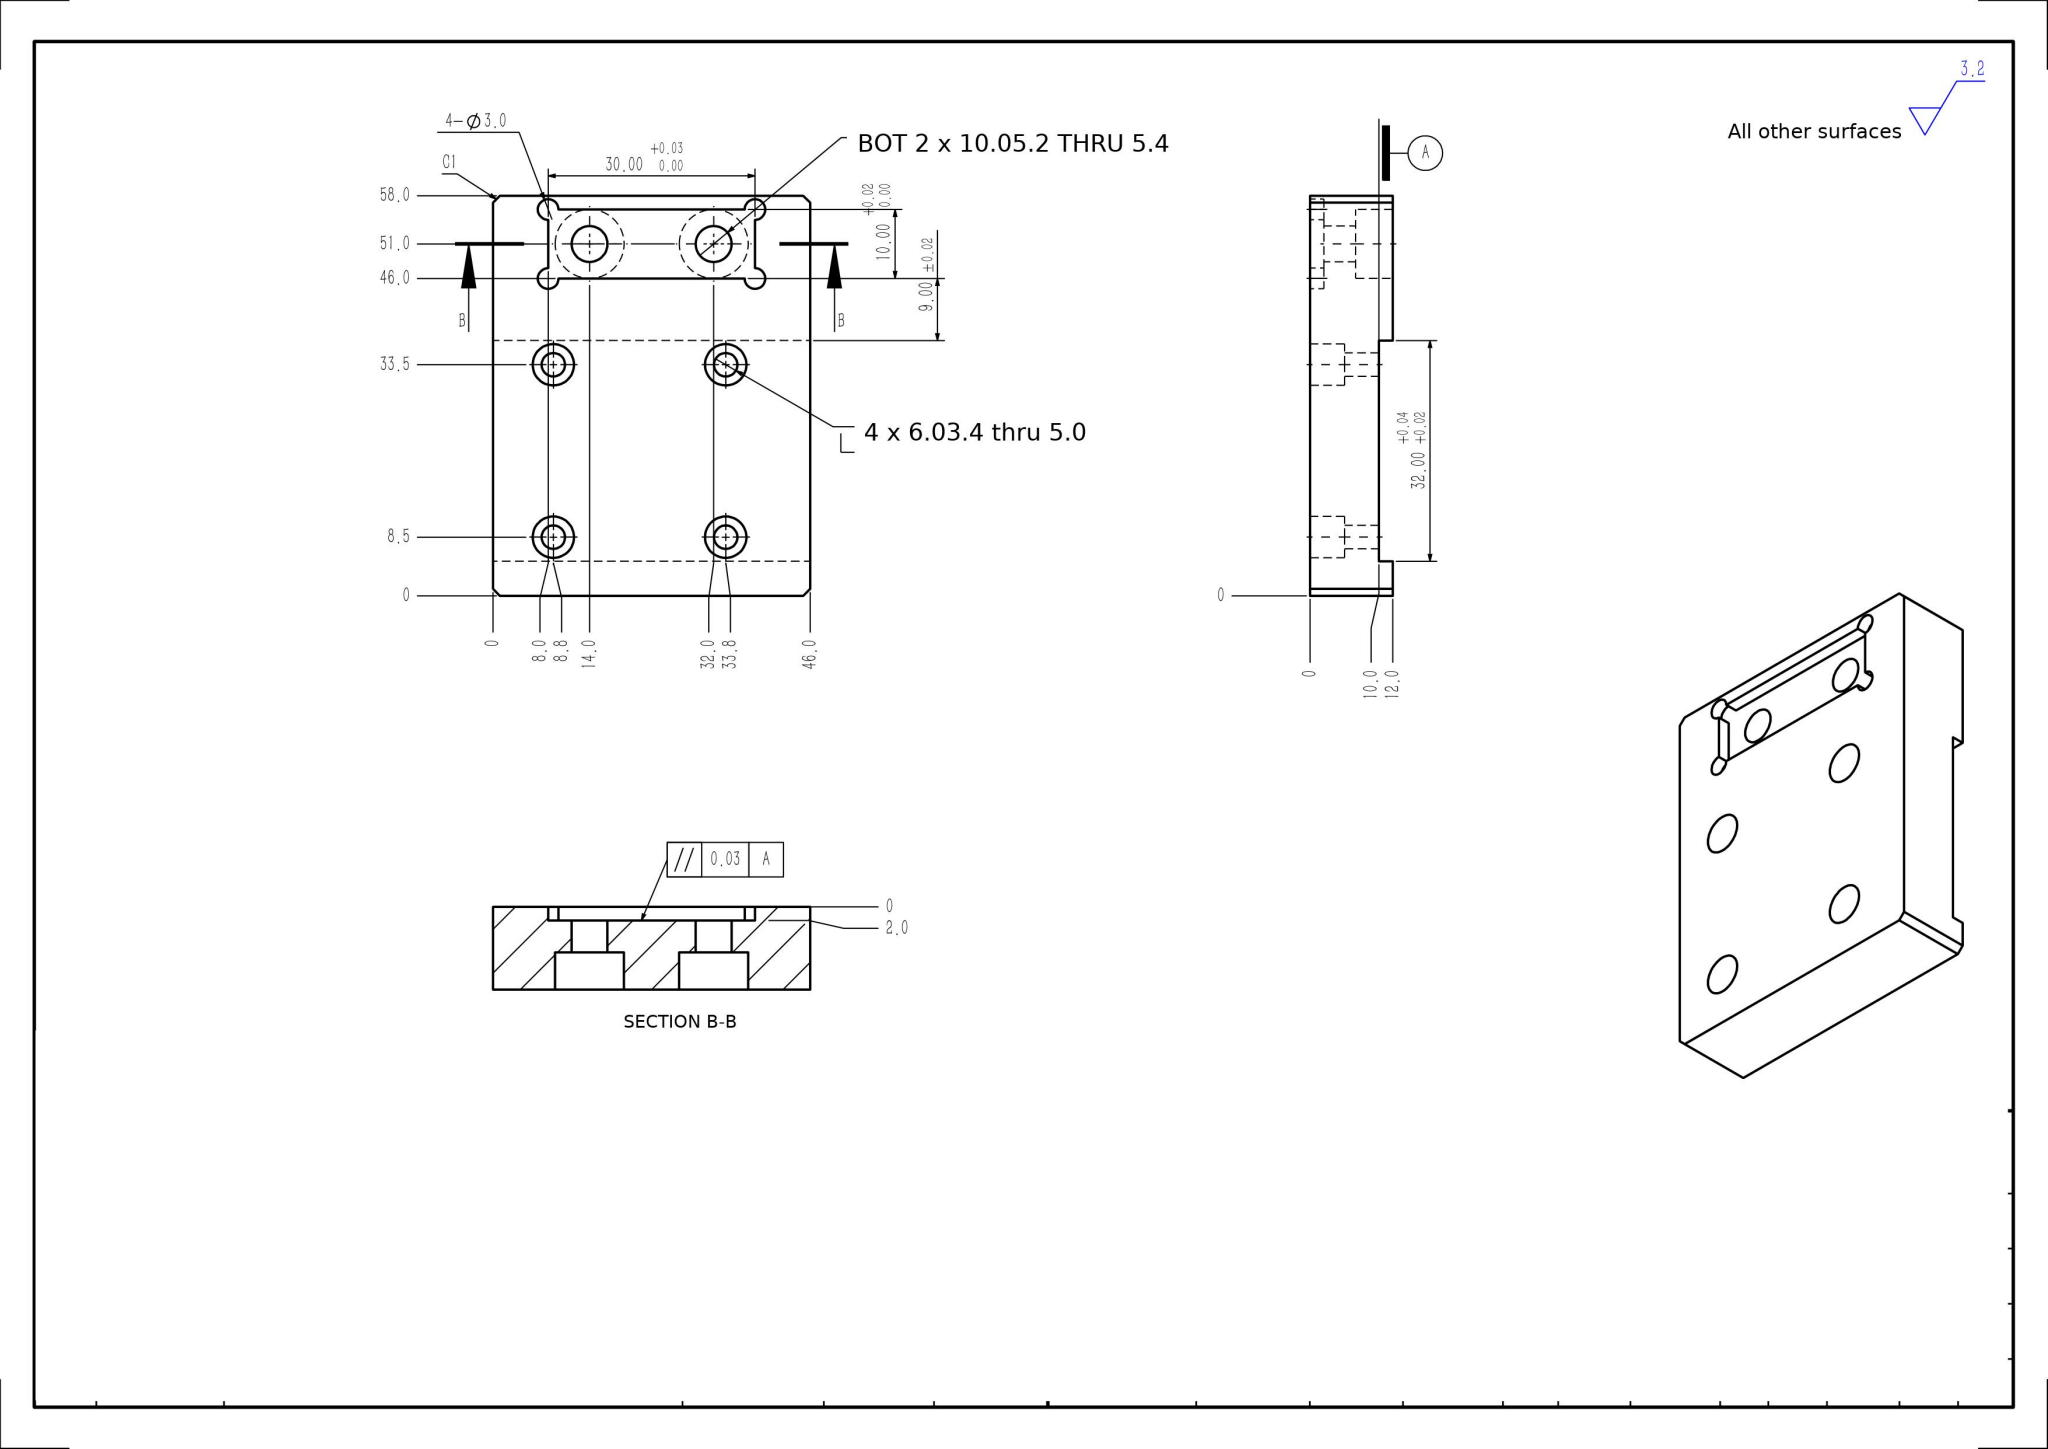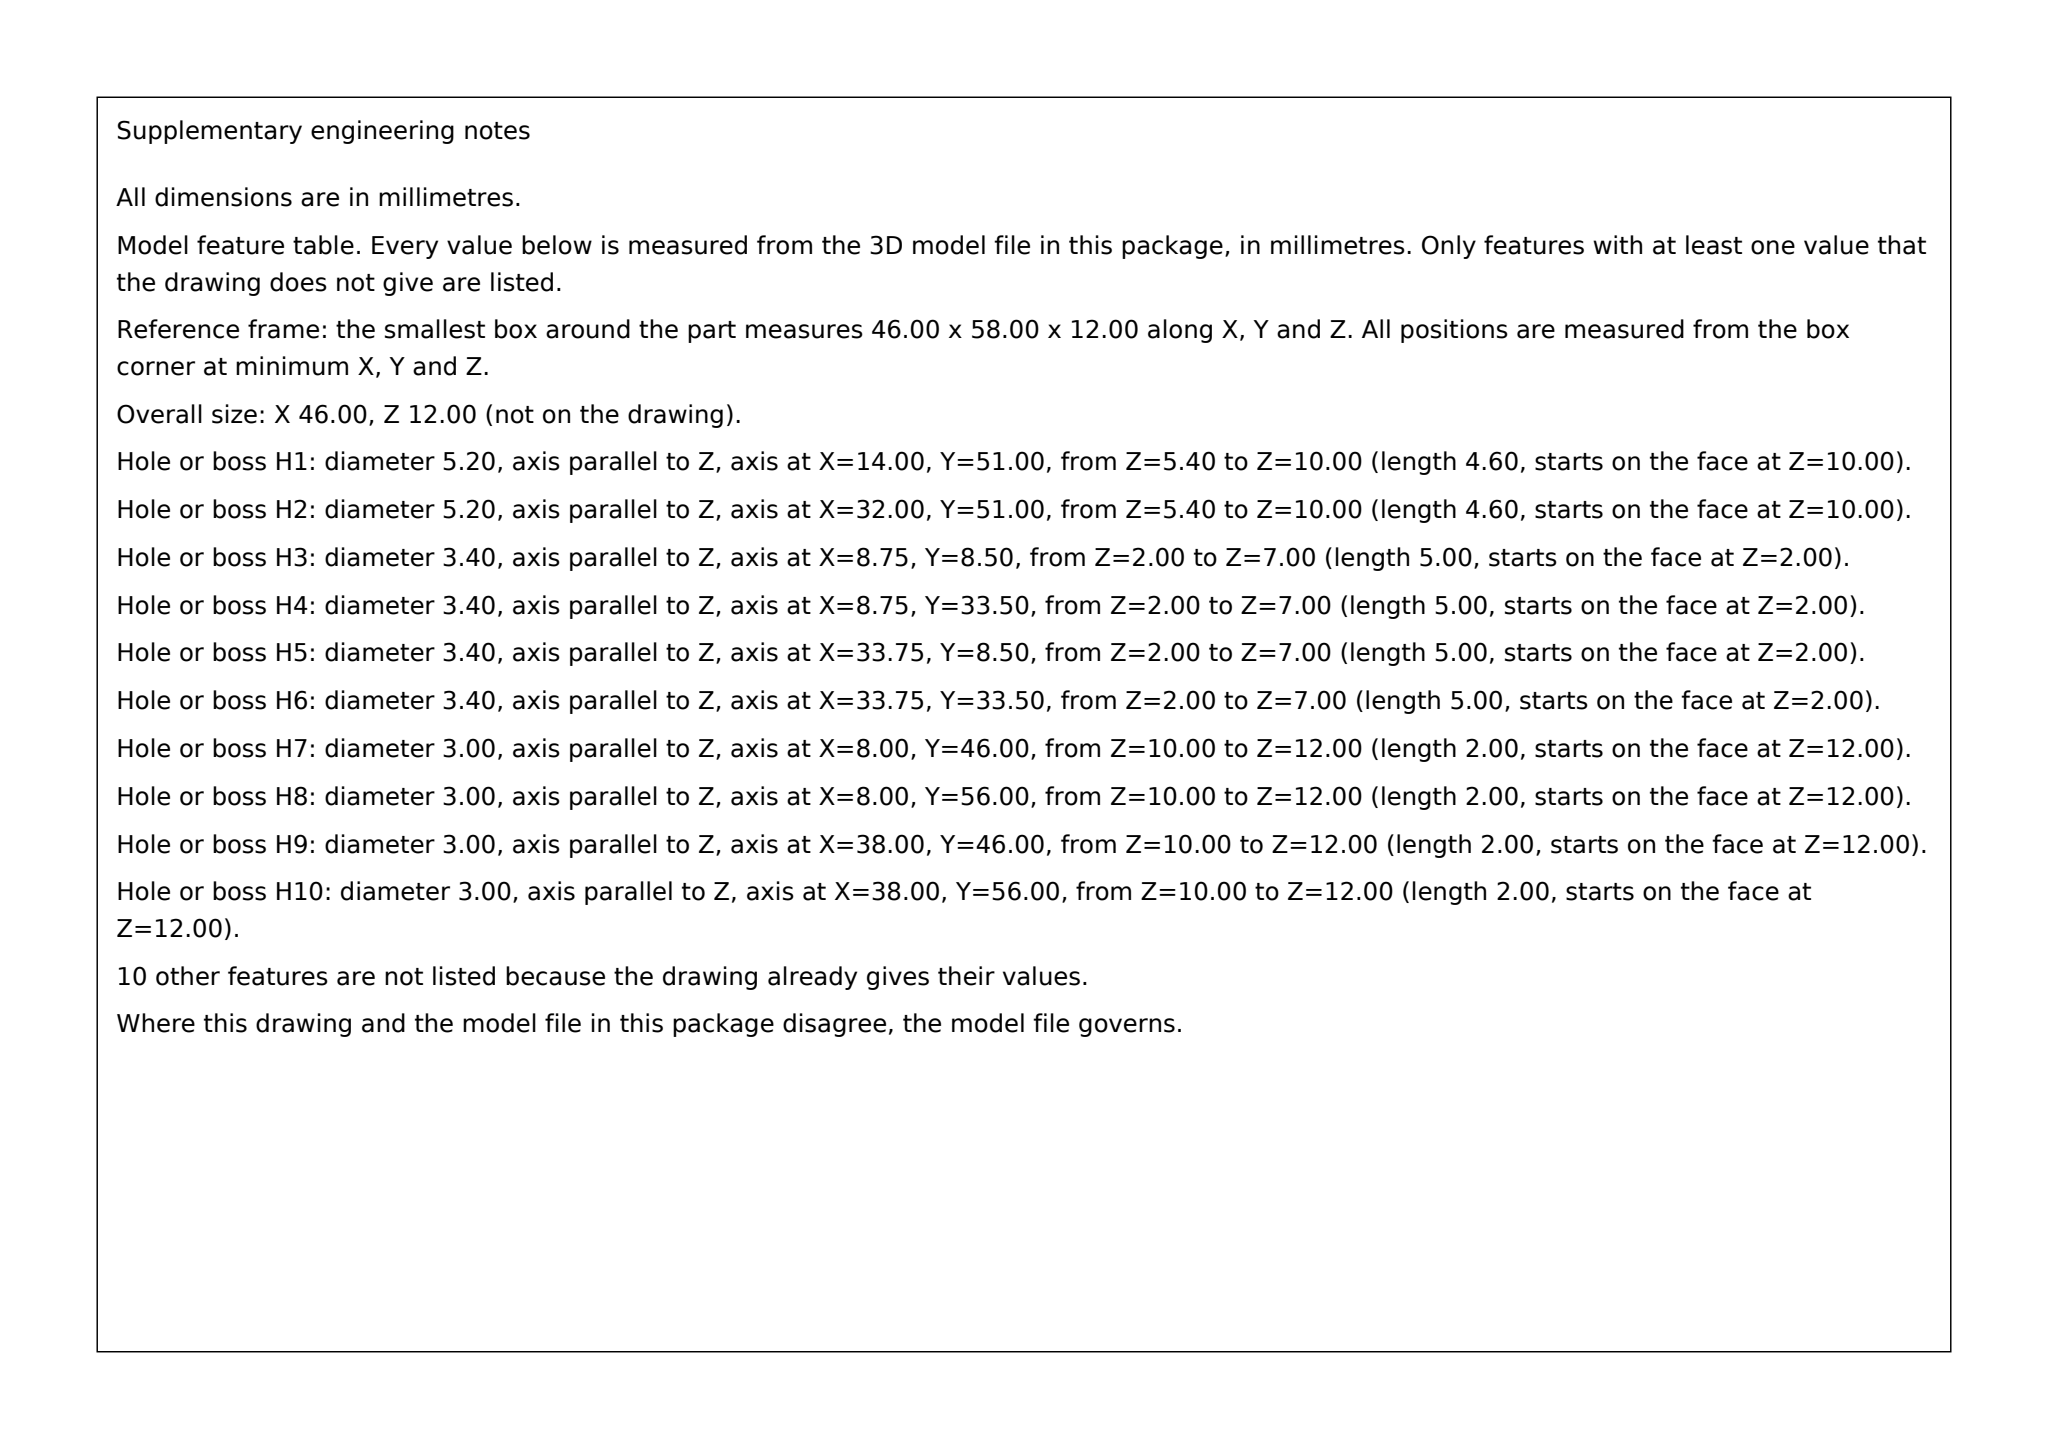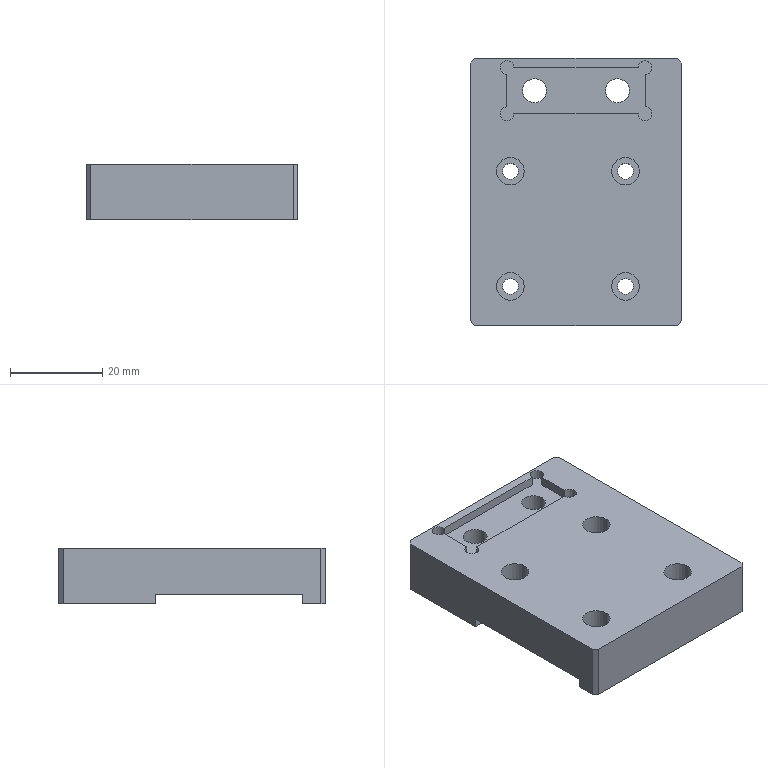Part | SolidWorks | mm | 1 solid | 55 faces | box 46 x 58 x 12 mm | volume 26615 mm3 | cylinder 30 | plane 25 | commonest cylinder face diameters 6 x8 3.4 x8 3 x6 10 x4 5.2 x4
build123d program:
from build123d import *

# Parameters (mm, degrees)
SKETCH1_W                                       = 46
SKETCH1_H                                       = 58
BOSS_EXTRUDE1_DEPTH                             = 12
SKETCH2_W                                       = 46
SKETCH2_H                                       = 32
CUT_EXTRUDE1_DEPTH                              = 2
M5_HEX_SOCKET_HEAD_CAP_SCREW_CBORE1_D           = 5.2
M5_HEX_SOCKET_HEAD_CAP_SCREW_CBORE1_CBORE_D     = 10
M5_HEX_SOCKET_HEAD_CAP_SCREW_CBORE1_CBORE_DEPTH = 5.4
SKETCH5_W                                       = 30
SKETCH5_H                                       = 10
CUT_EXTRUDE2_DEPTH                              = 2
SKETCH6_R                                       = 1.5
CUT_EXTRUDE3_DEPTH                              = 2
CHAMFER1_SIZE                                   = 1
M3_HEX_SOCKET_HEAD_CAP_SCREW_CBORE1_D           = 3.4
M3_HEX_SOCKET_HEAD_CAP_SCREW_CBORE1_CBORE_D     = 6
M3_HEX_SOCKET_HEAD_CAP_SCREW_CBORE1_CBORE_DEPTH = 5


with BuildPart() as part:
    # Sketch1 → Boss-Extrude1 (new body)
    with BuildSketch(Plane.XY):
        Rectangle(SKETCH1_W, SKETCH1_H)
    extrude(amount=BOSS_EXTRUDE1_DEPTH)

    # Sketch2 → Cut-Extrude1 (cut)
    with BuildSketch(Plane(origin=(0, 0, 0), x_dir=(-1, 0, 0), z_dir=(0, 0, -1))):
        with Locations((0, -8)):
            Rectangle(SKETCH2_W, SKETCH2_H)
    extrude(amount=-CUT_EXTRUDE1_DEPTH, mode=Mode.SUBTRACT)

    # M5 Hex Socket Head Cap Screw CBORE1 (through all)
    with Locations(Plane(origin=(0, 0, 0), x_dir=(-1, 0, 0), z_dir=(0, 0, -1))):
        with Locations((-9, 22), (9, 22)):
            CounterBoreHole(M5_HEX_SOCKET_HEAD_CAP_SCREW_CBORE1_D / 2, M5_HEX_SOCKET_HEAD_CAP_SCREW_CBORE1_CBORE_D / 2, M5_HEX_SOCKET_HEAD_CAP_SCREW_CBORE1_CBORE_DEPTH)

    # Sketch5 → Cut-Extrude2 (cut)
    with BuildSketch(Plane.XY.offset(12)):
        with Locations((0, 22)):
            Rectangle(SKETCH5_W, SKETCH5_H)
    extrude(amount=-CUT_EXTRUDE2_DEPTH, mode=Mode.SUBTRACT)

    # Sketch6 → Cut-Extrude3 (cut)
    with BuildSketch(Plane.XY.offset(12)):
        with Locations((15, 27)):
            Circle(SKETCH6_R)
        with Locations((-15, 27)):
            Circle(SKETCH6_R)
        with Locations((-15, 17)):
            Circle(SKETCH6_R)
        with Locations((15, 17)):
            Circle(SKETCH6_R)
    extrude(amount=-CUT_EXTRUDE3_DEPTH, mode=Mode.SUBTRACT)

    # Chamfer1
    chamfer1_edges = [part.edges().sort_by_distance(p)[0] for p in [
        (23, -29, 6),
        (-23, -29, 6),
        (-23, 29, 6),
        (23, 29, 6),
    ]]
    chamfer(chamfer1_edges, length=CHAMFER1_SIZE)

    # M3 Hex Socket Head Cap Screw CBORE1 (through all)
    with Locations(Plane.XY.offset(12)):
        with Locations((-14.25, 4.5), (-14.25, -20.5), (10.75, -20.5), (10.75, 4.5)):
            CounterBoreHole(M3_HEX_SOCKET_HEAD_CAP_SCREW_CBORE1_D / 2, M3_HEX_SOCKET_HEAD_CAP_SCREW_CBORE1_CBORE_D / 2, M3_HEX_SOCKET_HEAD_CAP_SCREW_CBORE1_CBORE_DEPTH)


solid = part.part